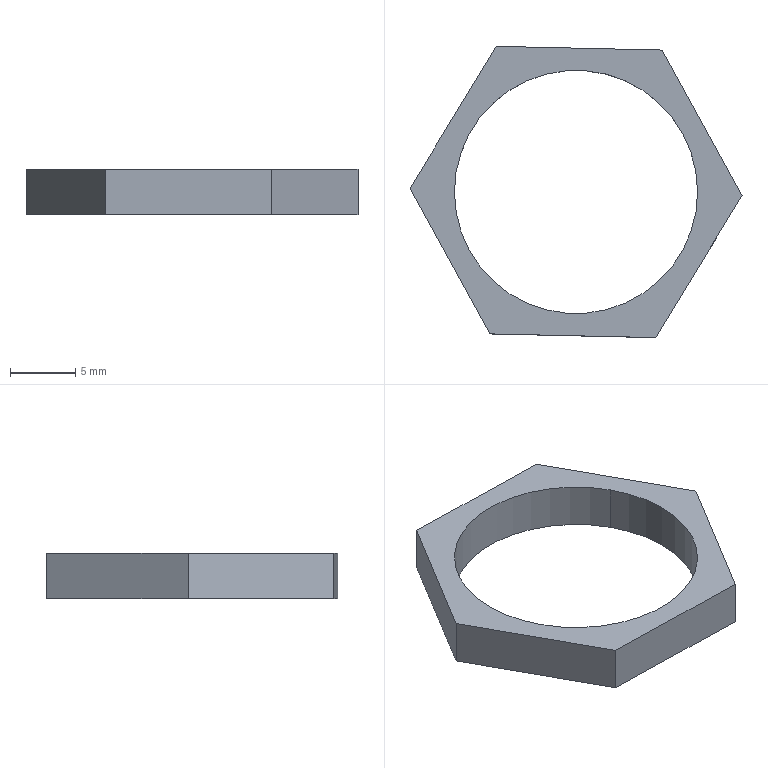Component | SolidWorks | PC-CAJ-P09-1_Tuerca Chapa Guantera Duesco-1 | 1 solid | 10 faces | box 25.4 x 22.28 x 3.5 mm | volume 516 mm3 | plane 8 | cylinder 2 | commonest cylinder face diameters 18.6 x2 | material Plain Carbon Steel
STEP:
#1=CARTESIAN_POINT('',(-0.3211,10.615,3.465));
#2=VERTEX_POINT('',#1);
#3=CARTESIAN_POINT('',(0.3211,10.967,3.465));
#4=VERTEX_POINT('',#3);
#5=CARTESIAN_POINT('',(-0.,10.791,3.465));
#6=DIRECTION('',(-0.,-0.,-1.));
#7=DIRECTION('',(0.8769,0.4806,-0.));
#8=AXIS2_PLACEMENT_3D('',#5,#6,#7);
#9=CIRCLE('',#8,0.3661);
#10=EDGE_CURVE('',#2,#4,#9,.T.);
#11=ORIENTED_EDGE('',*,*,#10,.F.);
#12=CARTESIAN_POINT('',(-0.3211,10.615,3.327));
#13=VERTEX_POINT('',#12);
#14=CARTESIAN_POINT('',(-0.3211,10.615,3.465));
#15=DIRECTION('',(-0.,-0.,-1.));
#16=VECTOR('',#15,39.37);
#17=LINE('',#14,#16);
#18=EDGE_CURVE('',#2,#13,#17,.T.);
#19=ORIENTED_EDGE('',*,*,#18,.T.);
#20=CARTESIAN_POINT('',(0.3211,10.967,3.327));
#21=VERTEX_POINT('',#20);
#22=CARTESIAN_POINT('',(-0.,10.791,3.327));
#23=DIRECTION('',(-0.,-0.,-1.));
#24=DIRECTION('',(0.8769,0.4806,-0.));
#25=AXIS2_PLACEMENT_3D('',#22,#23,#24);
#26=CIRCLE('',#25,0.3661);
#27=EDGE_CURVE('',#13,#21,#26,.T.);
#28=ORIENTED_EDGE('',*,*,#27,.T.);
#29=CARTESIAN_POINT('',(0.3211,10.967,3.465));
#30=DIRECTION('',(-0.,-0.,-1.));
#31=VECTOR('',#30,39.37);
#32=LINE('',#29,#31);
#33=EDGE_CURVE('',#4,#21,#32,.T.);
#34=ORIENTED_EDGE('',*,*,#33,.F.);
#35=EDGE_LOOP('',(#11,#19,#28,#34));
#36=FACE_OUTER_BOUND('',#35,.T.);
#37=CARTESIAN_POINT('',(-0.,10.791,3.465));
#38=DIRECTION('',(-0.,-0.,-1.));
#39=DIRECTION('',(0.8769,0.4806,-0.));
#40=AXIS2_PLACEMENT_3D('',#37,#38,#39);
#41=CYLINDRICAL_SURFACE('',#40,0.3661);
#42=ADVANCED_FACE('',(#36),#41,.F.);
#43=CARTESIAN_POINT('',(-0.,10.791,3.327));
#44=DIRECTION('',(-0.,-0.,-1.));
#45=DIRECTION('',(0.8769,0.4806,-0.));
#46=AXIS2_PLACEMENT_3D('',#43,#44,#45);
#47=CIRCLE('',#46,0.3661);
#48=EDGE_CURVE('',#21,#13,#47,.T.);
#49=ORIENTED_EDGE('',*,*,#48,.F.);
#50=ORIENTED_EDGE('',*,*,#27,.F.);
#51=EDGE_LOOP('',(#49,#50));
#52=FACE_BOUND('',#51,.T.);
#53=CARTESIAN_POINT('',(-0.2403,11.23,3.327));
#54=VERTEX_POINT('',#53);
#55=CARTESIAN_POINT('',(0.2596,11.219,3.327));
#56=VERTEX_POINT('',#55);
#57=CARTESIAN_POINT('',(-0.2403,11.23,3.327));
#58=DIRECTION('',(0.9998,-0.02227,0.));
#59=VECTOR('',#58,39.37);
#60=LINE('',#57,#59);
#61=EDGE_CURVE('',#54,#56,#60,.T.);
#62=ORIENTED_EDGE('',*,*,#61,.T.);
#63=CARTESIAN_POINT('',(0.4999,10.78,3.327));
#64=VERTEX_POINT('',#63);
#65=CARTESIAN_POINT('',(0.3798,10.999,3.327));
#66=DIRECTION('',(0.4806,-0.8769,0.));
#67=VECTOR('',#66,39.37);
#68=LINE('',#65,#67);
#69=EDGE_CURVE('',#56,#64,#68,.T.);
#70=ORIENTED_EDGE('',*,*,#69,.T.);
#71=CARTESIAN_POINT('',(0.2403,10.353,3.327));
#72=VERTEX_POINT('',#71);
#73=CARTESIAN_POINT('',(0.4999,10.78,3.327));
#74=DIRECTION('',(-0.5192,-0.8547,0.));
#75=VECTOR('',#74,39.37);
#76=LINE('',#73,#75);
#77=EDGE_CURVE('',#64,#72,#76,.T.);
#78=ORIENTED_EDGE('',*,*,#77,.T.);
#79=CARTESIAN_POINT('',(-0.2596,10.364,3.327));
#80=VERTEX_POINT('',#79);
#81=CARTESIAN_POINT('',(0.2403,10.353,3.327));
#82=DIRECTION('',(-0.9998,0.02227,-0.));
#83=VECTOR('',#82,39.37);
#84=LINE('',#81,#83);
#85=EDGE_CURVE('',#72,#80,#84,.T.);
#86=ORIENTED_EDGE('',*,*,#85,.T.);
#87=CARTESIAN_POINT('',(-0.4999,10.802,3.327));
#88=VERTEX_POINT('',#87);
#89=CARTESIAN_POINT('',(-0.3798,10.583,3.327));
#90=DIRECTION('',(-0.4806,0.8769,-0.));
#91=VECTOR('',#90,39.37);
#92=LINE('',#89,#91);
#93=EDGE_CURVE('',#80,#88,#92,.T.);
#94=ORIENTED_EDGE('',*,*,#93,.T.);
#95=CARTESIAN_POINT('',(-0.4999,10.802,3.327));
#96=DIRECTION('',(0.5192,0.8547,-0.));
#97=VECTOR('',#96,39.37);
#98=LINE('',#95,#97);
#99=EDGE_CURVE('',#88,#54,#98,.T.);
#100=ORIENTED_EDGE('',*,*,#99,.T.);
#101=EDGE_LOOP('',(#62,#70,#78,#86,#94,#100));
#102=FACE_OUTER_BOUND('',#101,.T.);
#103=CARTESIAN_POINT('',(-0.6201,11.022,3.327));
#104=DIRECTION('',(-0.,-0.,-1.));
#105=DIRECTION('',(0.8769,0.4806,-0.));
#106=AXIS2_PLACEMENT_3D('',#103,#104,#105);
#107=PLANE('',#106);
#108=ADVANCED_FACE('',(#52,#102),#107,.T.);
#109=CARTESIAN_POINT('',(-0.,10.791,3.465));
#110=DIRECTION('',(-0.,-0.,-1.));
#111=DIRECTION('',(0.8769,0.4806,-0.));
#112=AXIS2_PLACEMENT_3D('',#109,#110,#111);
#113=CIRCLE('',#112,0.3661);
#114=EDGE_CURVE('',#4,#2,#113,.T.);
#115=ORIENTED_EDGE('',*,*,#114,.T.);
#116=ORIENTED_EDGE('',*,*,#10,.T.);
#117=EDGE_LOOP('',(#115,#116));
#118=FACE_BOUND('',#117,.T.);
#119=CARTESIAN_POINT('',(-0.4999,10.802,3.465));
#120=VERTEX_POINT('',#119);
#121=CARTESIAN_POINT('',(-0.2596,10.364,3.465));
#122=VERTEX_POINT('',#121);
#123=CARTESIAN_POINT('',(-0.3798,10.583,3.465));
#124=DIRECTION('',(0.4806,-0.8769,0.));
#125=VECTOR('',#124,39.37);
#126=LINE('',#123,#125);
#127=EDGE_CURVE('',#120,#122,#126,.T.);
#128=ORIENTED_EDGE('',*,*,#127,.T.);
#129=CARTESIAN_POINT('',(0.2403,10.353,3.465));
#130=VERTEX_POINT('',#129);
#131=CARTESIAN_POINT('',(-0.2596,10.364,3.465));
#132=DIRECTION('',(0.9998,-0.02227,0.));
#133=VECTOR('',#132,39.37);
#134=LINE('',#131,#133);
#135=EDGE_CURVE('',#122,#130,#134,.T.);
#136=ORIENTED_EDGE('',*,*,#135,.T.);
#137=CARTESIAN_POINT('',(0.4999,10.78,3.465));
#138=VERTEX_POINT('',#137);
#139=CARTESIAN_POINT('',(0.2403,10.353,3.465));
#140=DIRECTION('',(0.5192,0.8547,-0.));
#141=VECTOR('',#140,39.37);
#142=LINE('',#139,#141);
#143=EDGE_CURVE('',#130,#138,#142,.T.);
#144=ORIENTED_EDGE('',*,*,#143,.T.);
#145=CARTESIAN_POINT('',(0.2596,11.219,3.465));
#146=VERTEX_POINT('',#145);
#147=CARTESIAN_POINT('',(0.3798,10.999,3.465));
#148=DIRECTION('',(-0.4806,0.8769,-0.));
#149=VECTOR('',#148,39.37);
#150=LINE('',#147,#149);
#151=EDGE_CURVE('',#138,#146,#150,.T.);
#152=ORIENTED_EDGE('',*,*,#151,.T.);
#153=CARTESIAN_POINT('',(-0.2403,11.23,3.465));
#154=VERTEX_POINT('',#153);
#155=CARTESIAN_POINT('',(0.2596,11.219,3.465));
#156=DIRECTION('',(-0.9998,0.02227,-0.));
#157=VECTOR('',#156,39.37);
#158=LINE('',#155,#157);
#159=EDGE_CURVE('',#146,#154,#158,.T.);
#160=ORIENTED_EDGE('',*,*,#159,.T.);
#161=CARTESIAN_POINT('',(-0.2403,11.23,3.465));
#162=DIRECTION('',(-0.5192,-0.8547,0.));
#163=VECTOR('',#162,39.37);
#164=LINE('',#161,#163);
#165=EDGE_CURVE('',#154,#120,#164,.T.);
#166=ORIENTED_EDGE('',*,*,#165,.T.);
#167=EDGE_LOOP('',(#128,#136,#144,#152,#160,#166));
#168=FACE_OUTER_BOUND('',#167,.T.);
#169=CARTESIAN_POINT('',(0.1395,11.438,3.465));
#170=DIRECTION('',(0.,0.,1.));
#171=DIRECTION('',(-0.8769,-0.4806,0.));
#172=AXIS2_PLACEMENT_3D('',#169,#170,#171);
#173=PLANE('',#172);
#174=ADVANCED_FACE('',(#118,#168),#173,.T.);
#175=CARTESIAN_POINT('',(0.2596,11.219,3.396));
#176=DIRECTION('',(0.,0.,1.));
#177=VECTOR('',#176,39.37);
#178=LINE('',#175,#177);
#179=EDGE_CURVE('',#56,#146,#178,.T.);
#180=ORIENTED_EDGE('',*,*,#179,.T.);
#181=ORIENTED_EDGE('',*,*,#151,.F.);
#182=CARTESIAN_POINT('',(0.4999,10.78,3.396));
#183=DIRECTION('',(-0.,-0.,-1.));
#184=VECTOR('',#183,39.37);
#185=LINE('',#182,#184);
#186=EDGE_CURVE('',#138,#64,#185,.T.);
#187=ORIENTED_EDGE('',*,*,#186,.T.);
#188=ORIENTED_EDGE('',*,*,#69,.F.);
#189=EDGE_LOOP('',(#180,#181,#187,#188));
#190=FACE_OUTER_BOUND('',#189,.T.);
#191=CARTESIAN_POINT('',(0.2596,11.219,3.465));
#192=DIRECTION('',(0.8769,0.4806,-0.));
#193=DIRECTION('',(0.4806,-0.8769,0.));
#194=AXIS2_PLACEMENT_3D('',#191,#192,#193);
#195=PLANE('',#194);
#196=ADVANCED_FACE('',(#190),#195,.T.);
#197=CARTESIAN_POINT('',(-0.2403,11.23,3.396));
#198=DIRECTION('',(0.,0.,1.));
#199=VECTOR('',#198,39.37);
#200=LINE('',#197,#199);
#201=EDGE_CURVE('',#54,#154,#200,.T.);
#202=ORIENTED_EDGE('',*,*,#201,.T.);
#203=ORIENTED_EDGE('',*,*,#159,.F.);
#204=ORIENTED_EDGE('',*,*,#179,.F.);
#205=ORIENTED_EDGE('',*,*,#61,.F.);
#206=EDGE_LOOP('',(#202,#203,#204,#205));
#207=FACE_OUTER_BOUND('',#206,.T.);
#208=CARTESIAN_POINT('',(-0.2403,11.23,3.465));
#209=DIRECTION('',(0.02227,0.9998,-0.));
#210=DIRECTION('',(0.9998,-0.02227,0.));
#211=AXIS2_PLACEMENT_3D('',#208,#209,#210);
#212=PLANE('',#211);
#213=ADVANCED_FACE('',(#207),#212,.T.);
#214=CARTESIAN_POINT('',(-0.4999,10.802,3.396));
#215=DIRECTION('',(0.,0.,1.));
#216=VECTOR('',#215,39.37);
#217=LINE('',#214,#216);
#218=EDGE_CURVE('',#88,#120,#217,.T.);
#219=ORIENTED_EDGE('',*,*,#218,.T.);
#220=ORIENTED_EDGE('',*,*,#165,.F.);
#221=ORIENTED_EDGE('',*,*,#201,.F.);
#222=ORIENTED_EDGE('',*,*,#99,.F.);
#223=EDGE_LOOP('',(#219,#220,#221,#222));
#224=FACE_OUTER_BOUND('',#223,.T.);
#225=CARTESIAN_POINT('',(-0.4999,10.802,3.465));
#226=DIRECTION('',(-0.8547,0.5192,-0.));
#227=DIRECTION('',(0.5192,0.8547,-0.));
#228=AXIS2_PLACEMENT_3D('',#225,#226,#227);
#229=PLANE('',#228);
#230=ADVANCED_FACE('',(#224),#229,.T.);
#231=CARTESIAN_POINT('',(-0.2596,10.364,3.396));
#232=DIRECTION('',(0.,0.,1.));
#233=VECTOR('',#232,39.37);
#234=LINE('',#231,#233);
#235=EDGE_CURVE('',#80,#122,#234,.T.);
#236=ORIENTED_EDGE('',*,*,#235,.T.);
#237=ORIENTED_EDGE('',*,*,#127,.F.);
#238=ORIENTED_EDGE('',*,*,#218,.F.);
#239=ORIENTED_EDGE('',*,*,#93,.F.);
#240=EDGE_LOOP('',(#236,#237,#238,#239));
#241=FACE_OUTER_BOUND('',#240,.T.);
#242=CARTESIAN_POINT('',(-0.2596,10.364,3.465));
#243=DIRECTION('',(-0.8769,-0.4806,0.));
#244=DIRECTION('',(-0.4806,0.8769,-0.));
#245=AXIS2_PLACEMENT_3D('',#242,#243,#244);
#246=PLANE('',#245);
#247=ADVANCED_FACE('',(#241),#246,.T.);
#248=CARTESIAN_POINT('',(0.2403,10.353,3.396));
#249=DIRECTION('',(0.,0.,1.));
#250=VECTOR('',#249,39.37);
#251=LINE('',#248,#250);
#252=EDGE_CURVE('',#72,#130,#251,.T.);
#253=ORIENTED_EDGE('',*,*,#252,.T.);
#254=ORIENTED_EDGE('',*,*,#135,.F.);
#255=ORIENTED_EDGE('',*,*,#235,.F.);
#256=ORIENTED_EDGE('',*,*,#85,.F.);
#257=EDGE_LOOP('',(#253,#254,#255,#256));
#258=FACE_OUTER_BOUND('',#257,.T.);
#259=CARTESIAN_POINT('',(0.2403,10.353,3.465));
#260=DIRECTION('',(-0.02227,-0.9998,0.));
#261=DIRECTION('',(-0.9998,0.02227,-0.));
#262=AXIS2_PLACEMENT_3D('',#259,#260,#261);
#263=PLANE('',#262);
#264=ADVANCED_FACE('',(#258),#263,.T.);
#265=ORIENTED_EDGE('',*,*,#186,.F.);
#266=ORIENTED_EDGE('',*,*,#143,.F.);
#267=ORIENTED_EDGE('',*,*,#252,.F.);
#268=ORIENTED_EDGE('',*,*,#77,.F.);
#269=EDGE_LOOP('',(#265,#266,#267,#268));
#270=FACE_OUTER_BOUND('',#269,.T.);
#271=CARTESIAN_POINT('',(0.4999,10.78,3.465));
#272=DIRECTION('',(0.8547,-0.5192,0.));
#273=DIRECTION('',(-0.5192,-0.8547,0.));
#274=AXIS2_PLACEMENT_3D('',#271,#272,#273);
#275=PLANE('',#274);
#276=ADVANCED_FACE('',(#270),#275,.T.);
#277=ORIENTED_EDGE('',*,*,#18,.F.);
#278=ORIENTED_EDGE('',*,*,#114,.F.);
#279=ORIENTED_EDGE('',*,*,#33,.T.);
#280=ORIENTED_EDGE('',*,*,#48,.T.);
#281=EDGE_LOOP('',(#277,#278,#279,#280));
#282=FACE_OUTER_BOUND('',#281,.T.);
#283=CARTESIAN_POINT('',(-0.,10.791,3.465));
#284=DIRECTION('',(-0.,-0.,-1.));
#285=DIRECTION('',(0.8769,0.4806,-0.));
#286=AXIS2_PLACEMENT_3D('',#283,#284,#285);
#287=CYLINDRICAL_SURFACE('',#286,0.3661);
#288=ADVANCED_FACE('',(#282),#287,.F.);
#289=CLOSED_SHELL('',(#42,#108,#174,#196,#213,#230,#247,#264,#276,#288));
#290=MANIFOLD_SOLID_BREP('',#289);
#291=CARTESIAN_POINT('',(0.,0.,0.));
#292=DIRECTION('',(0.,0.,1.));
#293=DIRECTION('',(1.,0.,0.));
#294=AXIS2_PLACEMENT_3D('',#291,#292,#293);
#295=(LENGTH_UNIT()NAMED_UNIT(*)SI_UNIT($,.METRE.));
#296=LENGTH_MEASURE_WITH_UNIT(LENGTH_MEASURE(0.0254),#295);
#297=DIMENSIONAL_EXPONENTS(1.,0.,0.,0.,0.,0.,0.);
#298=(CONVERSION_BASED_UNIT('',#296)LENGTH_UNIT()NAMED_UNIT(#297));
#299=UNCERTAINTY_MEASURE_WITH_UNIT(LENGTH_MEASURE(0.00001),#298,'','');
#300=(NAMED_UNIT(*)PLANE_ANGLE_UNIT()SI_UNIT($,.RADIAN.));
#301=(NAMED_UNIT(*)SI_UNIT($,.STERADIAN.)SOLID_ANGLE_UNIT());
#302=(GEOMETRIC_REPRESENTATION_CONTEXT(3)GLOBAL_UNCERTAINTY_ASSIGNED_CONTEXT((#299))GLOBAL_UNIT_ASSIGNED_CONTEXT((#298,#300,#301))REPRESENTATION_CONTEXT('',''));
#303=ADVANCED_BREP_SHAPE_REPRESENTATION('',(#290,#294),#302);
#304=COLOUR_RGB('',0.7922,0.8196,0.9333);
#305=FILL_AREA_STYLE_COLOUR('',#304);
#306=FILL_AREA_STYLE('',(#305));
#307=SURFACE_STYLE_FILL_AREA(#306);
#308=SURFACE_SIDE_STYLE('',(#307));
#309=SURFACE_STYLE_USAGE(.BOTH.,#308);
#310=PRESENTATION_STYLE_ASSIGNMENT((#309));
#311=STYLED_ITEM('',(#310),#290);
#312=(LENGTH_UNIT()NAMED_UNIT(*)SI_UNIT($,.METRE.));
#313=LENGTH_MEASURE_WITH_UNIT(LENGTH_MEASURE(0.0254),#312);
#314=DIMENSIONAL_EXPONENTS(1.,0.,0.,0.,0.,0.,0.);
#315=(CONVERSION_BASED_UNIT('',#313)LENGTH_UNIT()NAMED_UNIT(#314));
#316=UNCERTAINTY_MEASURE_WITH_UNIT(LENGTH_MEASURE(0.00001),#315,'','');
#317=(NAMED_UNIT(*)PLANE_ANGLE_UNIT()SI_UNIT($,.RADIAN.));
#318=(NAMED_UNIT(*)SI_UNIT($,.STERADIAN.)SOLID_ANGLE_UNIT());
#319=(GEOMETRIC_REPRESENTATION_CONTEXT(3)GLOBAL_UNCERTAINTY_ASSIGNED_CONTEXT((#316))GLOBAL_UNIT_ASSIGNED_CONTEXT((#315,#317,#318))REPRESENTATION_CONTEXT('',''));
#320=MECHANICAL_DESIGN_GEOMETRIC_PRESENTATION_REPRESENTATION('',(#311),#319);
#321=PRESENTATION_LAYER_ASSIGNMENT('','',(#311));